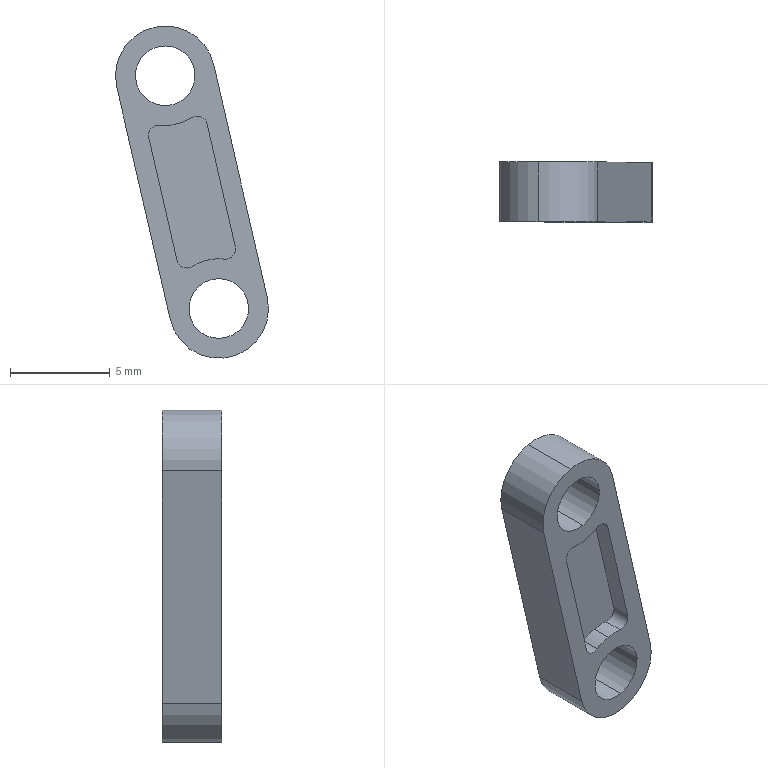Component | SolidWorks | JawOne-1 | 1 solid | 35 faces | box 7.69 x 3 x 16.69 mm | volume 154 mm3 | cylinder 25 | plane 10 | commonest cylinder face diameters 1 x12 5 x9 3 x4
build123d program:
from build123d import *

# Parameters (mm, degrees)
BOSS_EXTRUDE1_DEPTH  = 1.5
SKETCH2_R            = 1.5
CUT_EXTRUDE1_DEPTH   = 3
CUT_EXTRUDE2_DEPTH   = 1
FILLET1_R            = 0.5
FILLET1_OF_MIRROR1_R = 0.5


with BuildPart() as part:
    # Sketch1 → Boss-Extrude1 (new, symmetric)
    with BuildSketch(Plane.XY):
        with BuildLine():
            Line((-8, 2.5), (4, 2.5))
            ThreePointArc((4, 2.5), (6.5, 0), (4, -2.5))
            Line((4, -2.5), (-8, -2.5))
            ThreePointArc((-8, -2.5), (-10.5, 0), (-8, 2.5))
        make_face()
    extrude(amount=BOSS_EXTRUDE1_DEPTH, both=True)

    # Sketch2 → Cut-Extrude1 (cut)
    with BuildSketch(Plane.XY.offset(1.5)):
        with Locations((-8, 0)):
            Circle(SKETCH2_R)
        with Locations((4, 0)):
            Circle(SKETCH2_R)
    extrude(amount=-CUT_EXTRUDE1_DEPTH, mode=Mode.SUBTRACT)

    # Sketch3 → Cut-Extrude2 (cut)
    with BuildSketch(Plane.XY.offset(1.5)):
        with BuildLine():
            Line((2, 1.5), (-6, 1.5))
            ThreePointArc((-6, 1.5), (-5.5, 0), (-6, -1.5))
            Line((-6, -1.5), (2, -1.5))
            ThreePointArc((2, -1.5), (1.5, 0), (2, 1.5))
        make_face()
    cut_extrude2 = extrude(amount=-CUT_EXTRUDE2_DEPTH, mode=Mode.SUBTRACT)

    # Fillet1
    fillet1_edges = [part.edges().sort_by_distance(p)[0] for p in [
        (2, 1.5, 1),
        (2, -1.5, 1),
        (-6, -1.5, 1),
        (-6, 1.5, 1),
    ]]
    fillet(fillet1_edges, radius=FILLET1_R)

    # Mirror1: Cut-Extrude2 across plane
    add(cut_extrude2.mirror(Plane.XY), mode=Mode.SUBTRACT)

    # Fillet1 of Mirror1
    fillet1_of_mirror1_edges = [part.edges().sort_by_distance(p)[0] for p in [
        (2, 1.5, -1),
        (2, -1.5, -1),
        (-6, -1.5, -1),
        (-6, 1.5, -1),
    ]]
    fillet(fillet1_of_mirror1_edges, radius=FILLET1_OF_MIRROR1_R)


solid = part.part

# Placed as in the assembly
solid = solid.moved(Location((-24.071, -1.7, 220.11), (90, 0, -77.052)))